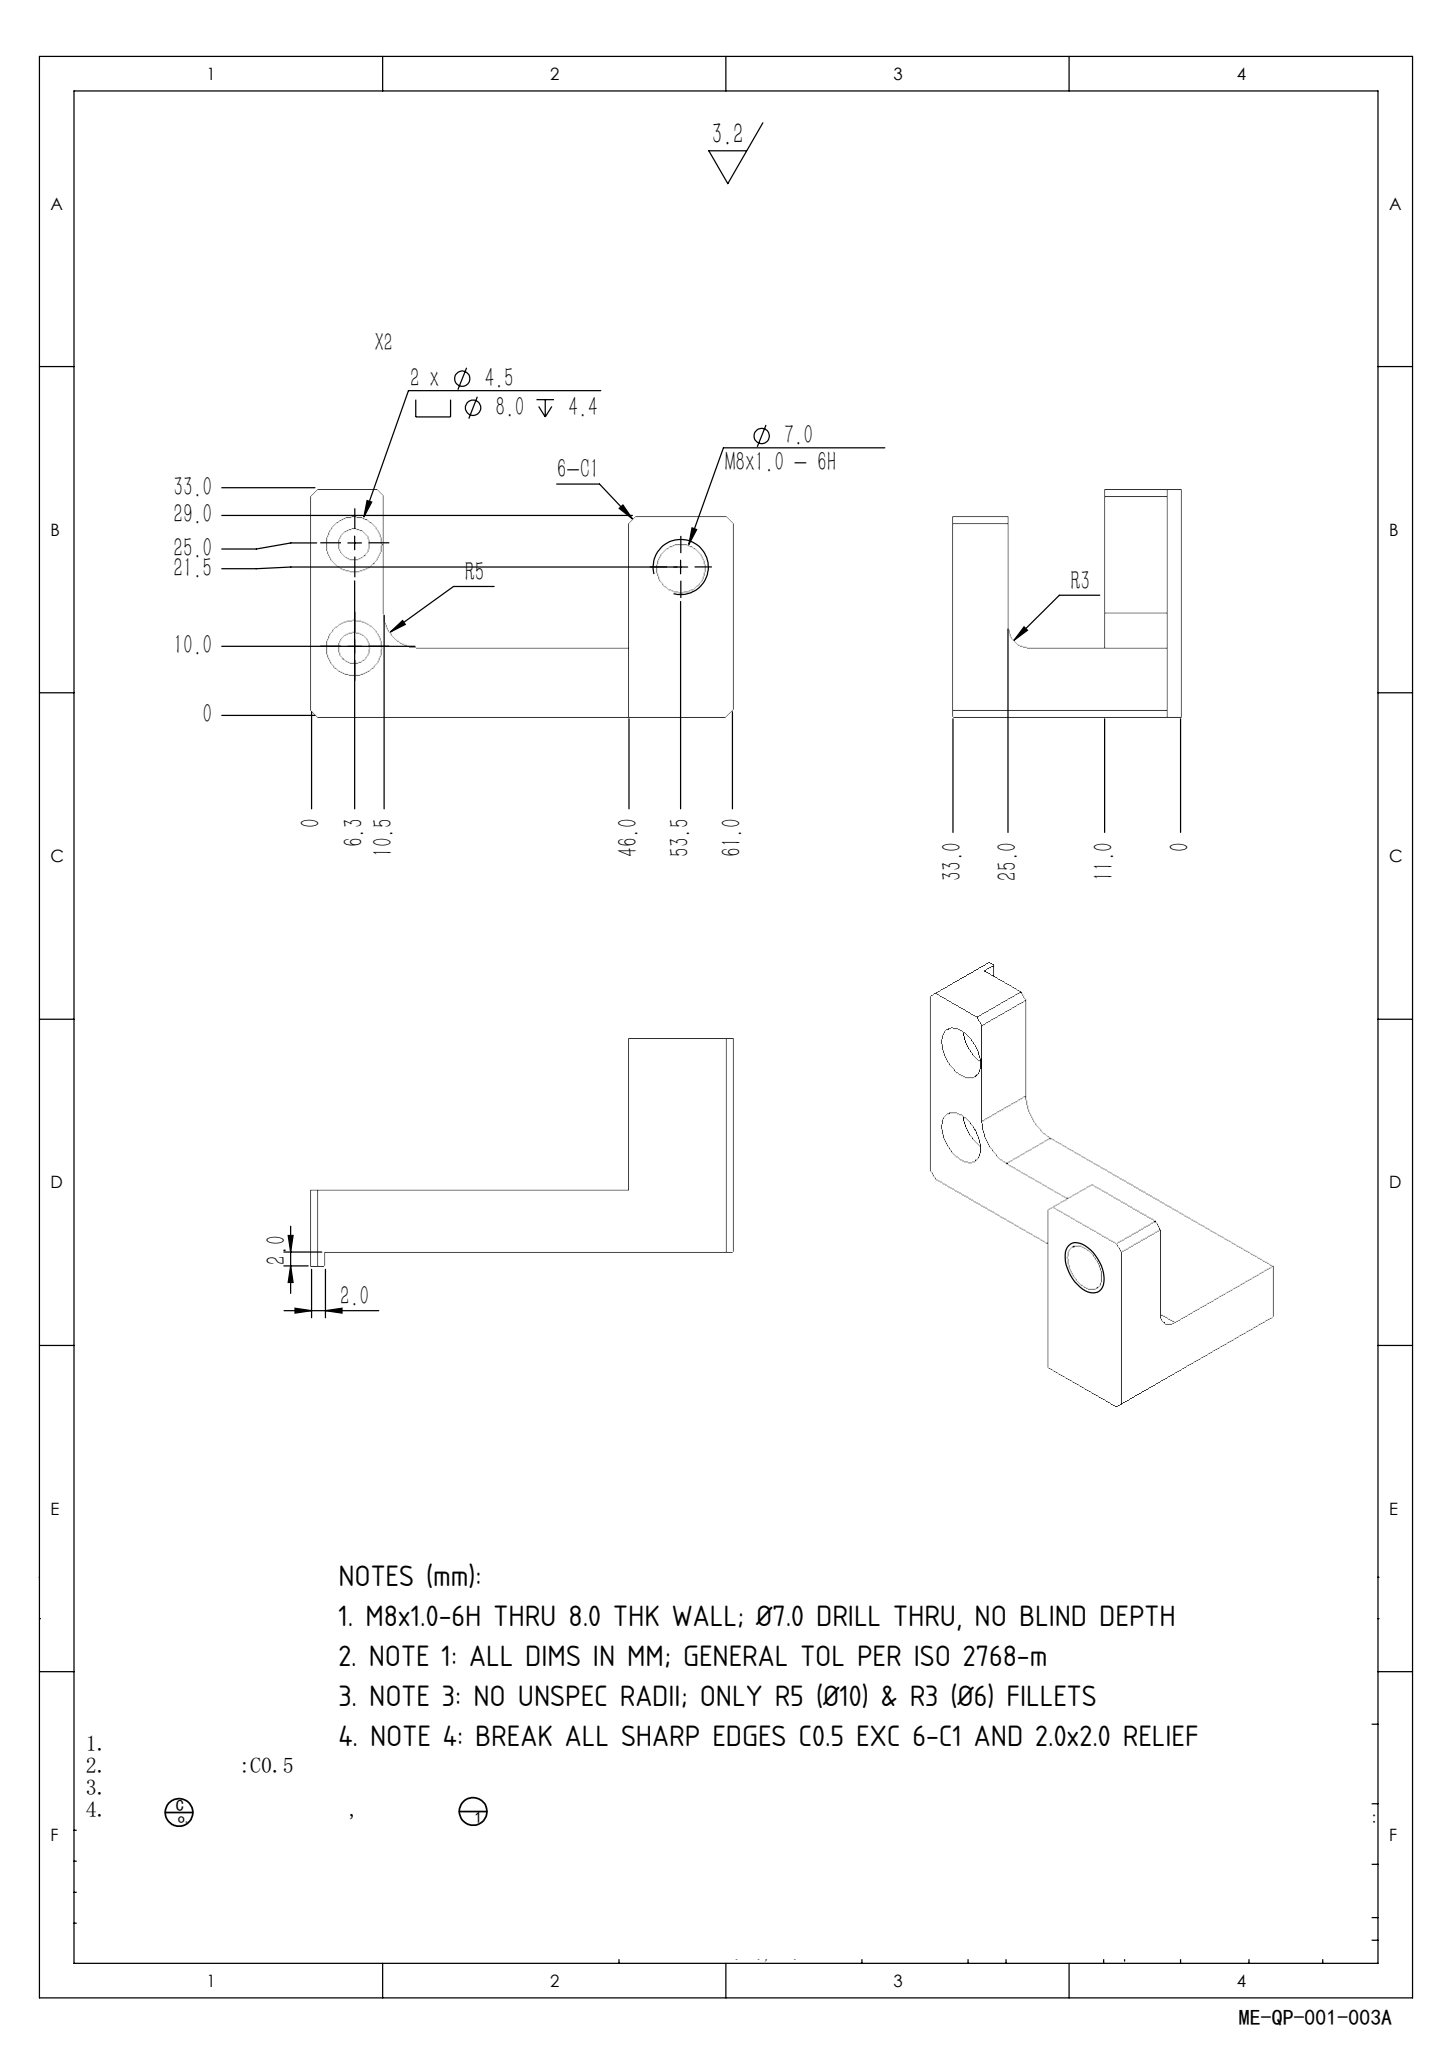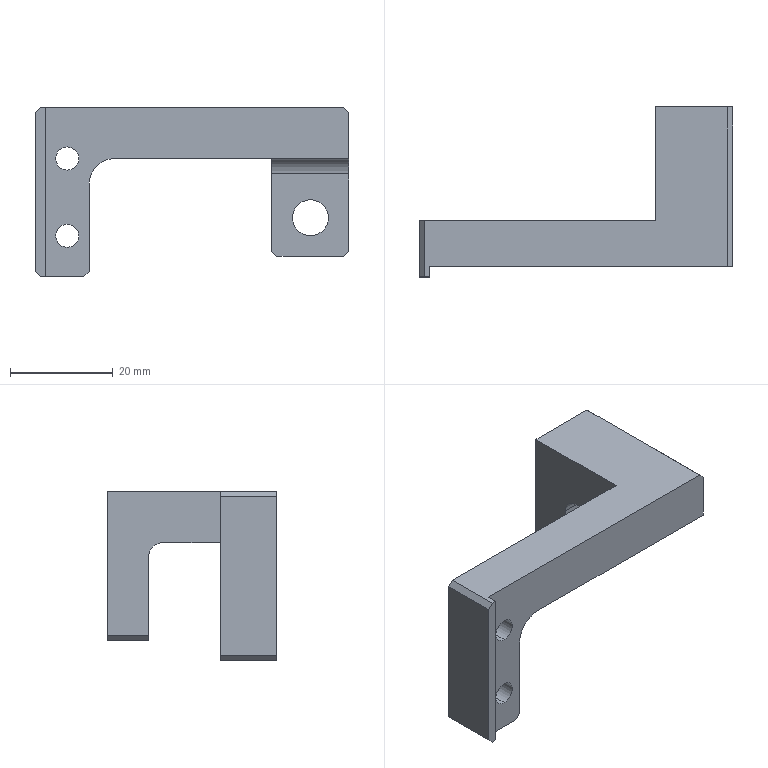Part | SolidWorks | mm | 1 solid | 34 faces | box 61 x 33 x 33 mm | volume 12517 mm3 | plane 22 | cylinder 12 | commonest cylinder face diameters 8 x4 4.5 x4 7 x2 10 x1 6 x1
Drawing notes:
M8x1.0-6H THRU 8.0 THK WALL; Ø7.0 DRILL THRU, NO BLIND DEPTH | from the solid: Ø7.0 cyl, axis Y at x=53.5, z=11.5, length 8.0; Y faces at 25.0 and 33.0 give 8.0 wall
NOTE 1: ALL DIMS IN MM; GENERAL TOL PER ISO 2768-m | from the solid: Model units mm, bbox 61.0 x 33.0 x 33.0; no toleranced features in STEP
NOTE 3: NO UNSPEC RADII; ONLY R5 (Ø10) & R3 (Ø6) FILLETS | from the solid: fillet_radii empty; Ø10.0 cyl axis Y at x=15.5,z=18.0 = R5; Ø6.0 cyl axis X at y=22.0,z=20.0 = R3
NOTE 4: BREAK ALL SHARP EDGES C0.5 EXC 6-C1 AND 2.0x2.0 RELIEF | from the solid: X planes 0.0/2.0 and Y planes 0.0/2.0 form the 2.0 x 2.0 relief; no other edge features in STEP